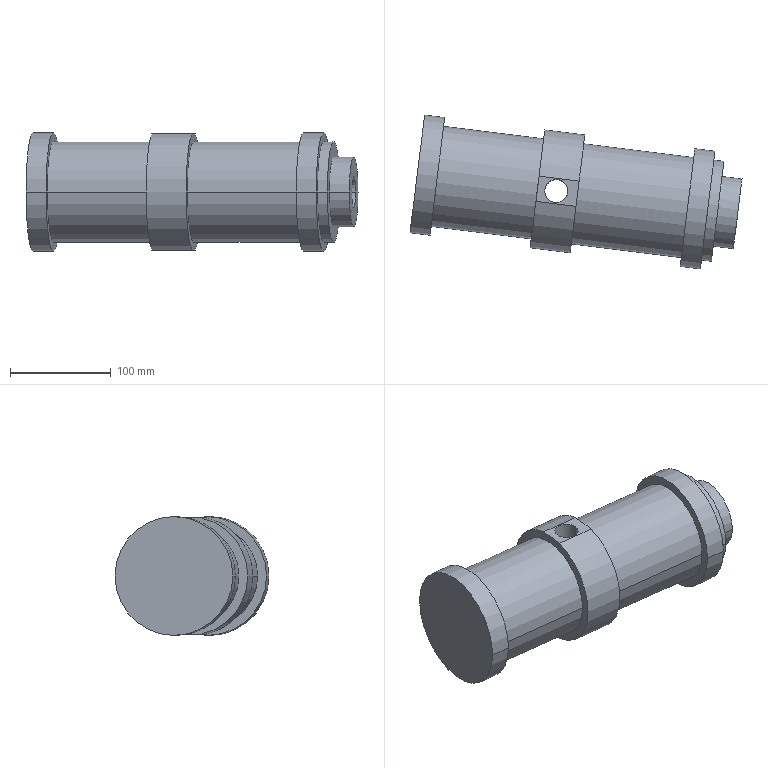Component | SolidWorks | Cylinder2-1 | 1 solid | 35 faces | box 329.12 x 152.63 x 117.71 mm | volume 2101100 mm3 | cylinder 23 | plane 12 | commonest cylinder face diameters 117.708 x7 100 x6 23 x4 50 x2 30 x2 69.715 x2
build123d program:
from build123d import *

# Parameters (mm, degrees)
SKETCH1_2_R                      = 50
BOSS_EXTRUDE1_DEPTH              = 300
SKETCH2_R                        = 25
CUT_EXTRUDE1_DEPTH               = 270
SKETCH3_R                        = 34.858
SKETCH3_R_2                      = 15
BOSS_EXTRUDE2_DEPTH              = 20
BOSS_EXTRUDE3_START              = -30
SKETCH4_R                        = 58.854
SKETCH4_R_2                      = 50
BOSS_EXTRUDE3_DEPTH              = 20
SKETCH5_2_R                      = 58.854
SKETCH5_2_R_2                    = 50
BOSS_EXTRUDE4_DEPTH              = 20
BOSS_EXTRUDE5_START              = -120
SKETCH5_2_2_R                    = 58.854
SKETCH5_2_2_R_2                  = 50
BOSS_EXTRUDE5_DEPTH              = 40
SKETCH6_R                        = 11.5
CUT_EXTRUDE2_DEPTH               = 90
TRUNNION_COLLAR_FLATS_DEPTH      = 40
TRUNNION_COLLAR_FLATS_DEPTH_BACK = 40
SKETCH1_W                        = 130
SKETCH1_H                        = 7.5


with BuildPart() as part:
    # Sketch1_2 → Boss-Extrude1 (new body)
    with BuildSketch(Plane.XY):
        Circle(SKETCH1_2_R)
    extrude(amount=BOSS_EXTRUDE1_DEPTH)

    # Sketch2 → Cut-Extrude1 (cut)
    with BuildSketch(Plane.XY.offset(300)):
        Circle(SKETCH2_R)
    extrude(amount=-CUT_EXTRUDE1_DEPTH, mode=Mode.SUBTRACT)

    # Sketch3 → Boss-Extrude2 (add)
    with BuildSketch(Plane.XY.offset(300)):
        Circle(SKETCH3_R)
        Circle(SKETCH3_R_2, mode=Mode.SUBTRACT)
    extrude(amount=BOSS_EXTRUDE2_DEPTH)

    # Sketch4 → Boss-Extrude3 (add)
    with BuildSketch(Plane.XY.offset(300).offset(BOSS_EXTRUDE3_START)):
        Circle(SKETCH4_R)
        Circle(SKETCH4_R_2, mode=Mode.SUBTRACT)
    extrude(amount=BOSS_EXTRUDE3_DEPTH)

    # Sketch5_2 → Boss-Extrude4 (add)
    with BuildSketch(Plane(origin=(0, 0, 0), x_dir=(-1, 0, 0), z_dir=(0, 0, -1))):
        with Locations(Location((0, 0, 0), (0, 0, 180))):
            Circle(SKETCH5_2_R)
        Circle(SKETCH5_2_R_2, mode=Mode.SUBTRACT)
    extrude(amount=-BOSS_EXTRUDE4_DEPTH)

    # Sketch5_2 2 → Boss-Extrude5 (add)
    with BuildSketch(Plane(origin=(0, 0, 0), x_dir=(-1, 0, 0), z_dir=(0, 0, -1)).offset(BOSS_EXTRUDE5_START)):
        with Locations(Location((0, 0, 0), (0, 0, 180))):
            Circle(SKETCH5_2_2_R)
        Circle(SKETCH5_2_2_R_2, mode=Mode.SUBTRACT)
    extrude(amount=-BOSS_EXTRUDE5_DEPTH)

    # Sketch6 → Cut-Extrude2 (cut, symmetric)
    with BuildSketch(Plane(origin=(0, 0, 0), x_dir=(1, 0, 0), z_dir=(0, 1, 0))):
        with Locations(Location((0, -138.772, 0), (0, 0, 270))):
            Circle(SKETCH6_R)
    extrude(amount=CUT_EXTRUDE2_DEPTH, both=True, mode=Mode.SUBTRACT)

    # Sketch1 → Trunnion collar flats (cut, two sides: drawn at the far end of the back side and taken through both)
    with BuildSketch(Plane(origin=(0, 0, 120), x_dir=(-1, 0, 0), z_dir=(0, 0, -1)).offset(-TRUNNION_COLLAR_FLATS_DEPTH_BACK)):
        with Locations((0, 61.25)):
            Rectangle(SKETCH1_W, SKETCH1_H)
        with Locations((0, -61.25)):
            Rectangle(SKETCH1_W, SKETCH1_H)
    extrude(amount=TRUNNION_COLLAR_FLATS_DEPTH + TRUNNION_COLLAR_FLATS_DEPTH_BACK, mode=Mode.SUBTRACT)


solid = part.part

# Placed as in the assembly
solid = solid.moved(Location((-152.709, -74.234, 495), (90, 82.905, 0)))